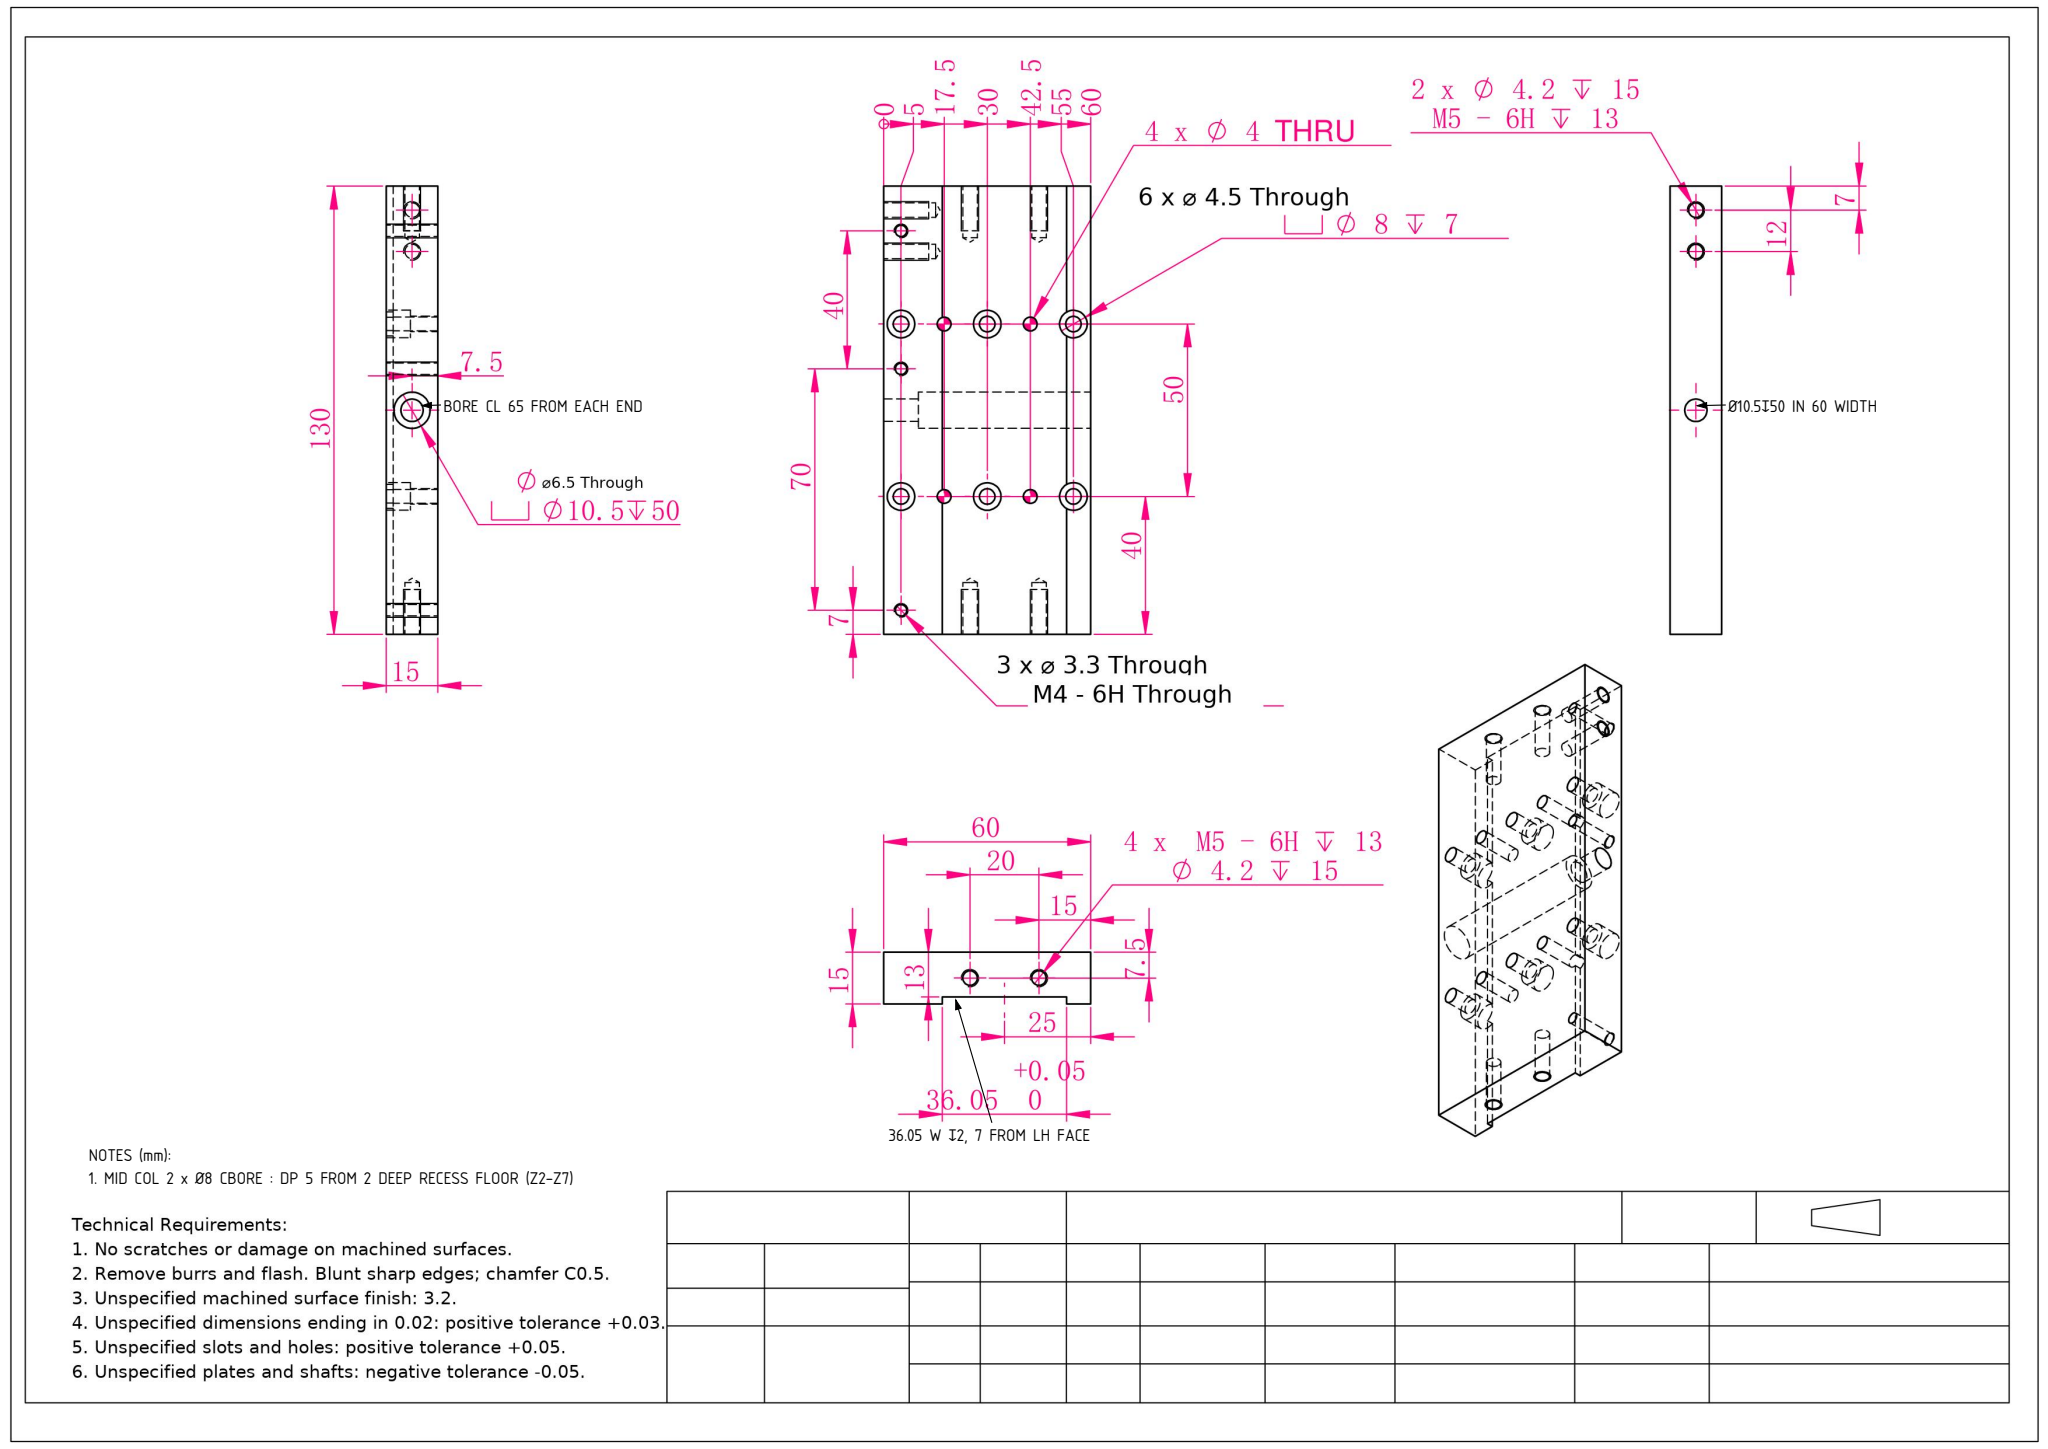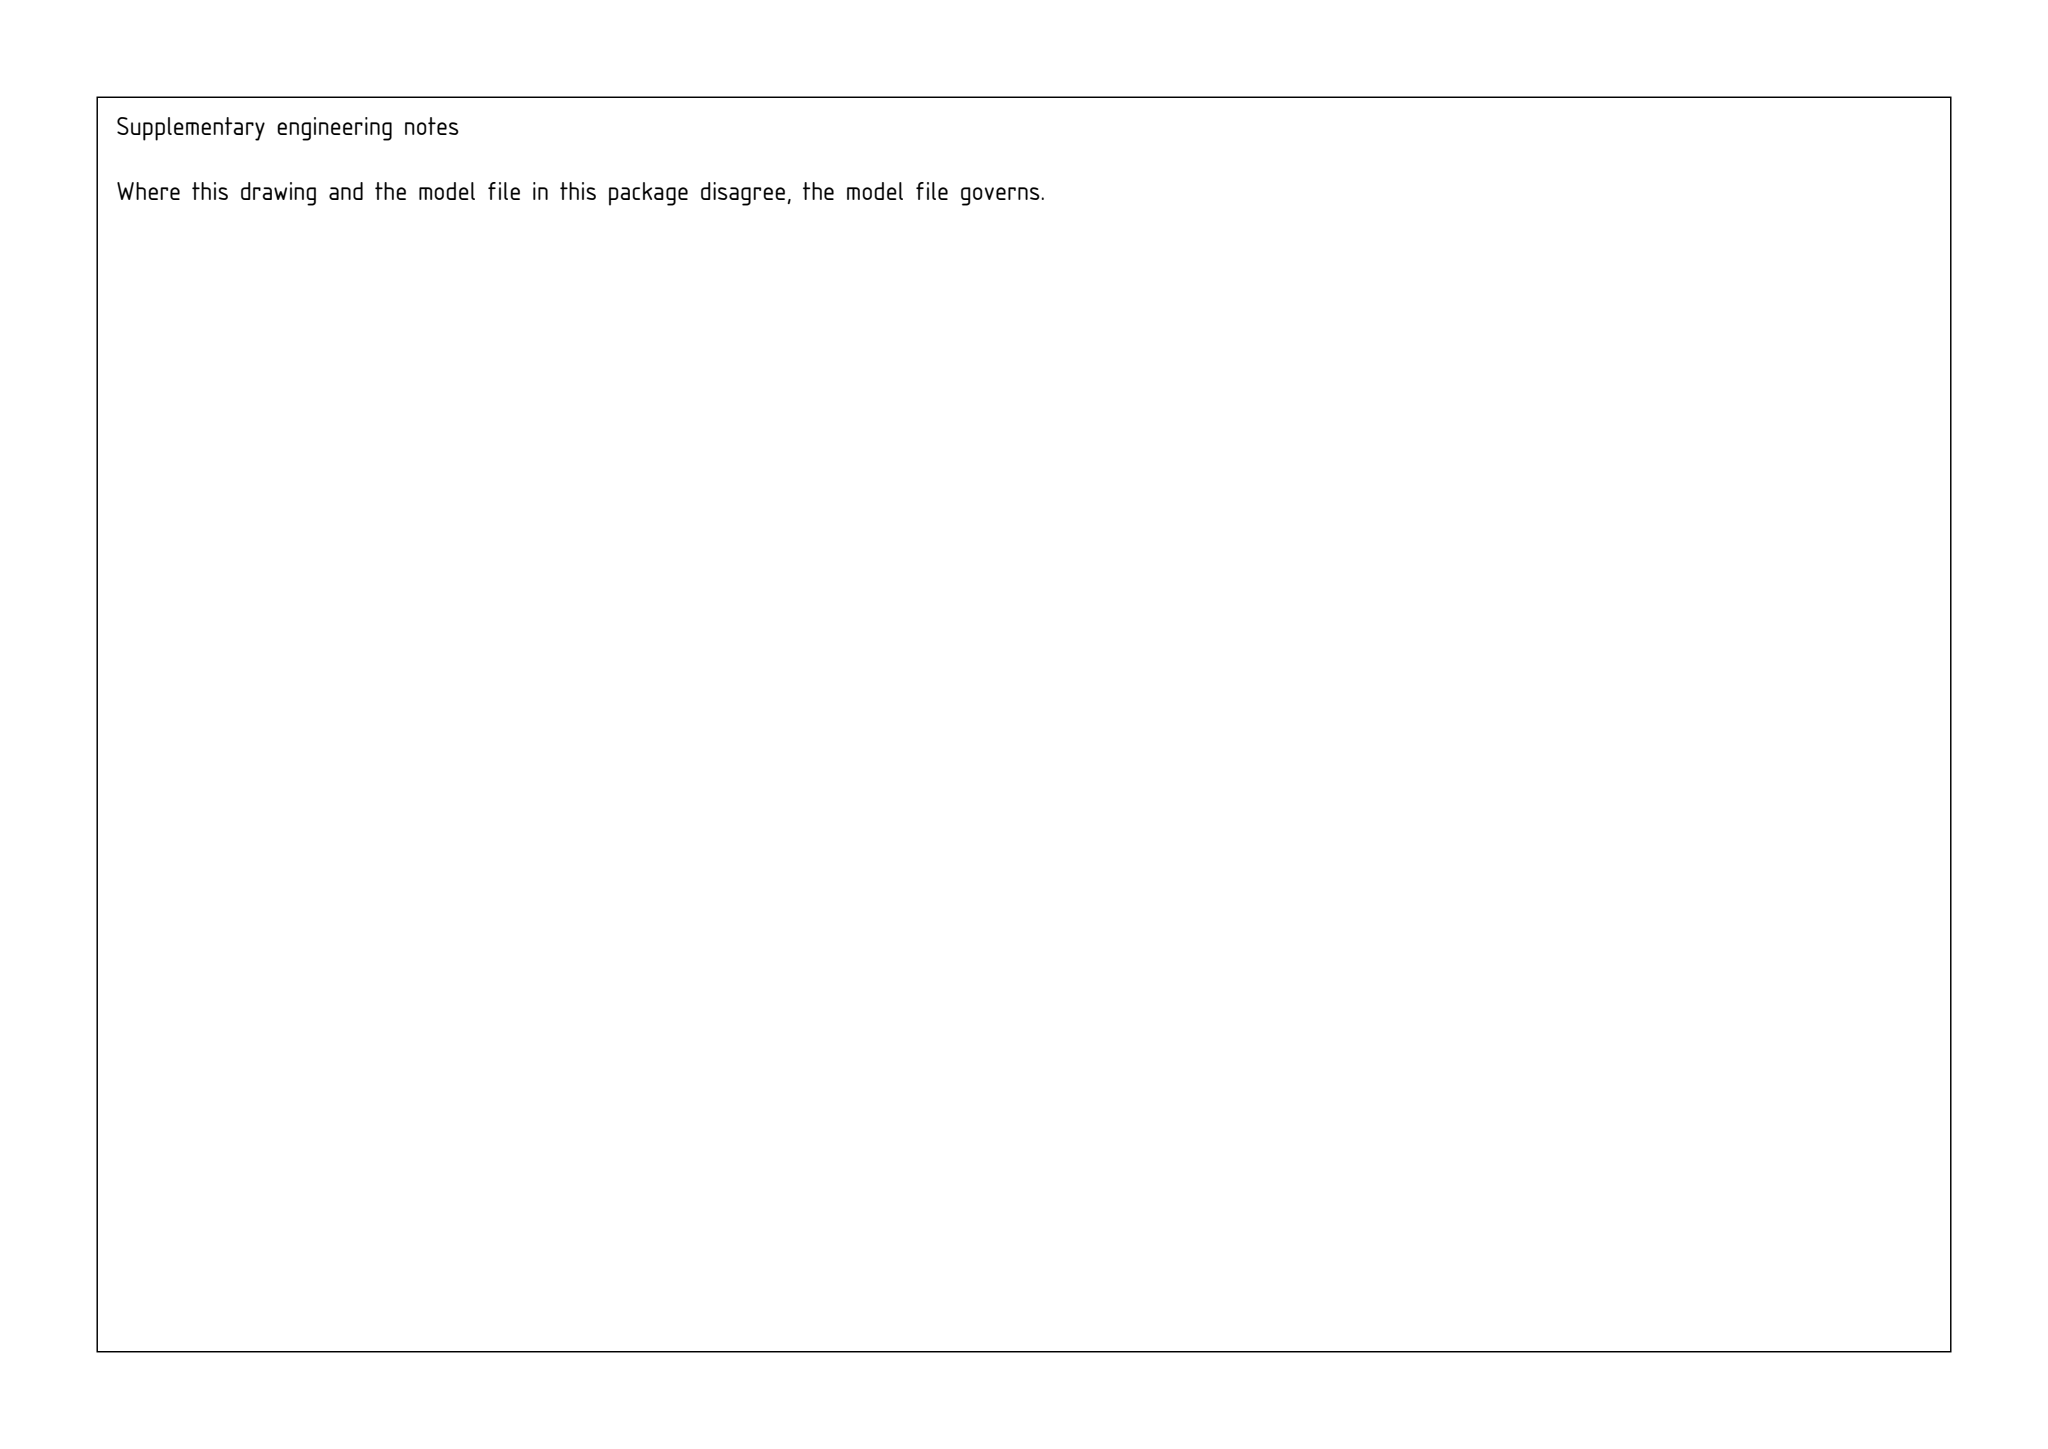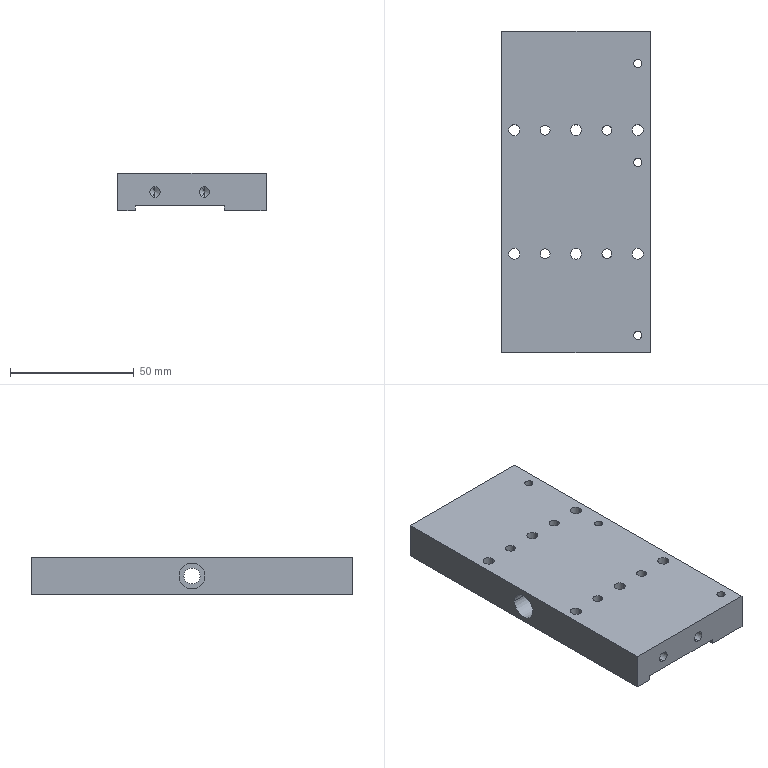Part | SolidWorks | mm | 1 solid | 87 faces | box 60 x 130 x 15 mm | volume 97995 mm3 | cylinder 54 | plane 21 | cone 12 | commonest cylinder face diameters 4.2 x12 8 x12 4.5 x12 4 x8 3.3 x6 10.5 x2 6.5 x2
Drawing notes:
BOTTOM RECESS 36.05 W x 2 DP: 7 FROM LH FACE, 17 FROM RH FACE | from the solid: z=2.0 floor plane extent x[7.0,43.0] over y[0,130]; z=0 faces x[0,7] & x[43,60]; part width 60
Ø6.5/Ø10.5 BORE CL 65 FROM EACH END - CL OF 130 | from the solid: Ø10.5 & Ø6.5 bores, axis x, y=65.0 of 130.0 length (mid-length)
MID COL 2 x Ø8 CBORE : DP 5 FROM 2 DEEP RECESS FLOOR (Z2-Z7) | from the solid: Ø8 bores at x=30, y=40/90 run z 2.0->7.0; recess floor plane z=2.0, x 7-43
Ø10.5 DP 50 IN 60 WIDTH (NOT 15 THK), THEN Ø6.5 THRU 10 | from the solid: Ø10.5 axis x from 0.0 to 50.0; Ø6.5 axis x from 50.0 to 60.0; bbox x=60
build123d program:
from build123d import *

# Parameters (mm, degrees)
SKETCH1_W                                       = 60
SKETCH1_H                                       = 130
BOSS_EXTRUDE1_DEPTH                             = 15
SKETCH7_R                                       = 3.25
CUT_EXTRUDE2_DEPTH                              = 20
SKETCH8_R                                       = 3.25
CUT_EXTRUDE3_DEPTH                              = 90.722
SKETCH11_R                                      = 5.25
CUT_EXTRUDE4_DEPTH                              = 50
M4_HEX_SOCKET_HEAD_CAP_SCREW_CBORE2_D           = 4.5
M4_HEX_SOCKET_HEAD_CAP_SCREW_CBORE2_CBORE_D     = 8
M4_HEX_SOCKET_HEAD_CAP_SCREW_CBORE2_CBORE_DEPTH = 7
SIZE_MM_DOWEL_PIN_HOLE_1_D                      = 4
SKETCH16_W                                      = 36.05
SKETCH16_H                                      = 130
CUT_EXTRUDE5_DEPTH                              = 2
M5_TAPPED_HOLE3_AT_2_COUNT                      = 2
M5_TAPPED_HOLE3_AT_2_PITCH                      = 20
M5_TAPPED_HOLE4_D                               = 4.2
M5_TAPPED_HOLE4_DEPTH                           = 15
M5_TAPPED_HOLE4_TIP                             = 1.262
M4_TAPPED_HOLE1_D                               = 3.3


with BuildPart() as part:
    # Sketch1 → Boss-Extrude1 (new body)
    with BuildSketch(Plane.XY):
        Rectangle(SKETCH1_W, SKETCH1_H)
    extrude(amount=BOSS_EXTRUDE1_DEPTH)

    # Sketch7 → Cut-Extrude2 (cut)
    with BuildSketch(Plane.ZY.offset(30)):
        with Locations(Location((7.5, 0, 0), (0, 0, 270))):
            Circle(SKETCH7_R)
    extrude(amount=-CUT_EXTRUDE2_DEPTH, mode=Mode.SUBTRACT)

    # Sketch8 → Cut-Extrude3 (cut, through all)
    with BuildSketch(Plane.ZY.offset(30)):
        with Locations(Location((7.5, 0, 0), (0, 0, 270))):
            Circle(SKETCH8_R)
    extrude(amount=-CUT_EXTRUDE3_DEPTH, mode=Mode.SUBTRACT)

    # Sketch11 → Cut-Extrude4 (cut)
    with BuildSketch(Plane.ZY.offset(30)):
        with Locations(Location((7.5, 0, 0), (0, 0, 270))):
            Circle(SKETCH11_R)
    extrude(amount=-CUT_EXTRUDE4_DEPTH, mode=Mode.SUBTRACT)

    # M4 Hex Socket Head Cap Screw CBORE2 (through all)
    with Locations(Plane(origin=(0, 0, 0), x_dir=(-1, 0, 0), z_dir=(0, 0, -1))):
        with Locations((25, 25), (0, 25), (-25, 25), (25, -25), (0, -25), (-25, -25)):
            CounterBoreHole(M4_HEX_SOCKET_HEAD_CAP_SCREW_CBORE2_D / 2, M4_HEX_SOCKET_HEAD_CAP_SCREW_CBORE2_CBORE_D / 2, M4_HEX_SOCKET_HEAD_CAP_SCREW_CBORE2_CBORE_DEPTH)

    # Size mm Dowel Pin Hole 1 (through all)
    with Locations(Plane(origin=(0, 0, 0), x_dir=(-1, 0, 0), z_dir=(0, 0, -1))):
        with Locations((12.5, 25), (-12.5, 25), (-12.5, -25), (12.5, -25)):
            Hole(SIZE_MM_DOWEL_PIN_HOLE_1_D / 2)

    # Sketch16 → Cut-Extrude5 (cut)
    with BuildSketch(Plane(origin=(0, 0, 0), x_dir=(-1, 0, 0), z_dir=(0, 0, -1))):
        with Locations((5, 0)):
            Rectangle(SKETCH16_W, SKETCH16_H)
    extrude(amount=-CUT_EXTRUDE5_DEPTH, mode=Mode.SUBTRACT)

    # Sketch19 → M5 Tapped Hole3 (revolve, cut)
    with BuildSketch(Plane(origin=(-15, 65, 7.5), x_dir=(0, 0, 1), z_dir=(1, 0, 0))):
        Polygon((0, 0), (0, 16.262), (2.1, 15), (2.1, 0), align=None)
    m5_tapped_hole3 = revolve(axis=Axis((-15, 71.35, 7.5), (0, -1, 0)), mode=Mode.SUBTRACT)

    # M5 Tapped Hole3 at 2: M5 Tapped Hole3 ×2
    with Locations(*[(i * M5_TAPPED_HOLE3_AT_2_PITCH, 0, 0) for i in range(1, M5_TAPPED_HOLE3_AT_2_COUNT)]):
        add(m5_tapped_hole3, mode=Mode.SUBTRACT)

    # Mirror1: M5 Tapped Hole3 across plane
    add(m5_tapped_hole3.mirror(Plane.ZX), mode=Mode.SUBTRACT)

    # Mirror1 copy 1 sketch → Mirror1 copy 1 (revolve, cut)
    with BuildSketch(Plane(origin=(5, -65, 7.5), x_dir=(0, 0, 1), z_dir=(1, 0, 0))):
        Polygon((0, 0), (0, -16.262), (2.1, -15), (2.1, 0), align=None)
    revolve(axis=Axis((5, -71.35, 7.5), (0, -1, 0)), mode=Mode.SUBTRACT)

    # M5 Tapped Hole4
    with Locations(Plane(origin=(30, 0, 0), x_dir=(0, 0, -1), z_dir=(1, 0, 0))):
        with Locations((-7.5, 46), (-7.5, 58)):
            Hole(M5_TAPPED_HOLE4_D / 2, depth=M5_TAPPED_HOLE4_DEPTH)
            with Locations((0, 0, -(M5_TAPPED_HOLE4_DEPTH + M5_TAPPED_HOLE4_TIP / 2))):  # 118° drill point
                Cone(0, M5_TAPPED_HOLE4_D / 2, M5_TAPPED_HOLE4_TIP, mode=Mode.SUBTRACT)

    # M4 Tapped Hole1 (through all)
    with Locations(Plane(origin=(0, 0, 0), x_dir=(-1, 0, 0), z_dir=(0, 0, -1))):
        with Locations((-25, 52), (-25, 12), (-25, -58)):
            Hole(M4_TAPPED_HOLE1_D / 2)


solid = part.part